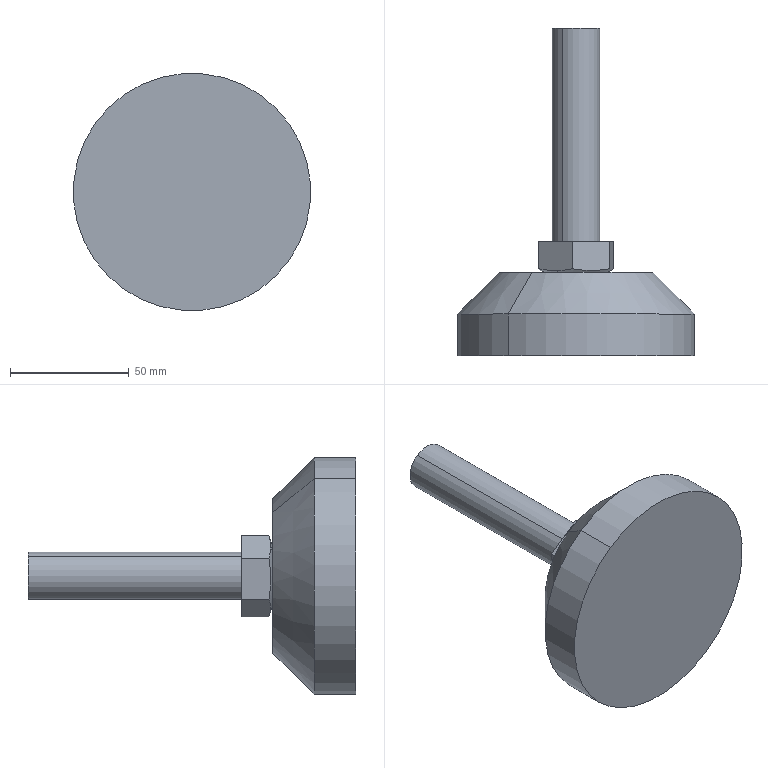Component | SolidWorks | 30-01A-1_Wheel-322-1_FBR100-20-322-1_pad1100-20-100pad1-322-1 | 1 solid | 23 faces | box 100 x 138 x 100 mm | volume 270529 mm3 | plane 11 | cylinder 8 | cone 4 | commonest cylinder face diameters 100 x2 57 x2 65 x2 20 x2
build123d program:
from build123d import *

# Parameters (mm, degrees)
SKETCH2_W          = 60
SKETCH2_H          = 60
CUT_EXTRUDE1_DEPTH = 14
SKETCH3_R          = 32.5
SKETCH3_R_2        = 28.5
CUT_EXTRUDE2_DEPTH = 0.1
SKETCH4_R          = 28.245
CUT_EXTRUDE3_DEPTH = 10


with BuildPart() as part:
    # Sketch1 → Revolve1 (revolve)
    with BuildSketch(Plane.XY, mode=Mode.PRIVATE) as revolve1_sk:
        Polygon((0, 148), (8.647, 148), (10, 146.647), (10, 48), (18.75, 48), (18.75, 37), (12, 35), (32.5, 35), (50, 17.5), (50, 0), (0, 0), align=None)
    revolve(revolve1_sk.sketch.rotate(Axis((0, 0, 0), (0, 1, 0)), 270), axis=Axis((0, 0, 0), (0, 1, 0)))

    # Sketch2 → Cut-Extrude1 (cut)
    with BuildSketch(Plane(origin=(0, 35, 0), x_dir=(-1, 0, 0), z_dir=(0, 1, 0))):
        Rectangle(SKETCH2_W, SKETCH2_H)
        Polygon((17.321, 0), (8.66, 15), (-8.66, 15), (-17.321, 0), (-8.66, -15), (8.66, -15), align=None, mode=Mode.SUBTRACT)
    extrude(amount=CUT_EXTRUDE1_DEPTH, mode=Mode.SUBTRACT)

    # Sketch3 → Cut-Extrude2 (cut)
    with BuildSketch(Plane(origin=(0, 35, 0), x_dir=(-1, 0, 0), z_dir=(0, 1, 0))):
        with Locations(Location((0, 0, 0), (0, 0, 90))):
            Circle(SKETCH3_R)
        with Locations(Location((0, 0, 0), (0, 0, 90))):
            Circle(SKETCH3_R_2, mode=Mode.SUBTRACT)
    extrude(amount=-CUT_EXTRUDE2_DEPTH, mode=Mode.SUBTRACT)

    # Sketch4 → Cut-Extrude3 (cut)
    with BuildSketch(Plane(origin=(0, 148, 0), x_dir=(1, 0, 0), z_dir=(0, 1, 0))):
        Circle(SKETCH4_R)
    extrude(amount=-CUT_EXTRUDE3_DEPTH, mode=Mode.SUBTRACT)


solid = part.part

# Placed as in the assembly
solid = solid.moved(Location((232.57, -660.845, -20), (180, 34.797, 180)))
STEP:
#1=CARTESIAN_POINT('',(9.886,-24.64,-1.838));
#2=VERTEX_POINT('',#1);
#3=CARTESIAN_POINT('',(8.426,-24.64,0.2633));
#4=VERTEX_POINT('',#3);
#5=CARTESIAN_POINT('',(9.156,-24.64,-0.7874));
#6=DIRECTION('',(0.,1.,-0.));
#7=DIRECTION('',(0.5707,0.,-0.8212));
#8=AXIS2_PLACEMENT_3D('',#5,#6,#7);
#9=CIRCLE('',#8,1.28);
#10=EDGE_CURVE('',#2,#4,#9,.T.);
#11=ORIENTED_EDGE('',*,*,#10,.F.);
#12=CARTESIAN_POINT('',(10.28,-25.329,-2.404));
#13=VERTEX_POINT('',#12);
#14=CARTESIAN_POINT('',(10.28,-25.329,-2.404));
#15=DIRECTION('',(0.4035,-0.7071,-0.5807));
#16=VECTOR('',#15,39.37);
#17=LINE('',#14,#16);
#18=EDGE_CURVE('',#2,#13,#17,.T.);
#19=ORIENTED_EDGE('',*,*,#18,.T.);
#20=CARTESIAN_POINT('',(8.033,-25.329,0.8291));
#21=VERTEX_POINT('',#20);
#22=CARTESIAN_POINT('',(9.156,-25.329,-0.7874));
#23=DIRECTION('',(0.,1.,-0.));
#24=DIRECTION('',(0.5707,0.,-0.8212));
#25=AXIS2_PLACEMENT_3D('',#22,#23,#24);
#26=CIRCLE('',#25,1.969);
#27=EDGE_CURVE('',#13,#21,#26,.T.);
#28=ORIENTED_EDGE('',*,*,#27,.T.);
#29=CARTESIAN_POINT('',(8.033,-25.329,0.8291));
#30=DIRECTION('',(-0.4035,-0.7071,0.5807));
#31=VECTOR('',#30,39.37);
#32=LINE('',#29,#31);
#33=EDGE_CURVE('',#4,#21,#32,.T.);
#34=ORIENTED_EDGE('',*,*,#33,.F.);
#35=EDGE_LOOP('',(#11,#19,#28,#34));
#36=FACE_OUTER_BOUND('',#35,.T.);
#37=CARTESIAN_POINT('',(9.156,-25.329,-0.7874));
#38=DIRECTION('',(-0.,-1.,0.));
#39=DIRECTION('',(-0.5707,0.,0.8212));
#40=AXIS2_PLACEMENT_3D('',#37,#38,#39);
#41=CONICAL_SURFACE('',#40,1.969,0.7854);
#42=ADVANCED_FACE('',(#36),#41,.T.);
#43=CARTESIAN_POINT('',(10.28,-26.018,-2.404));
#44=VERTEX_POINT('',#43);
#45=CARTESIAN_POINT('',(8.033,-26.018,0.8291));
#46=VERTEX_POINT('',#45);
#47=CARTESIAN_POINT('',(9.156,-26.018,-0.7874));
#48=DIRECTION('',(0.,1.,-0.));
#49=DIRECTION('',(0.5707,0.,-0.8212));
#50=AXIS2_PLACEMENT_3D('',#47,#48,#49);
#51=CIRCLE('',#50,1.969);
#52=EDGE_CURVE('',#44,#46,#51,.T.);
#53=ORIENTED_EDGE('',*,*,#52,.T.);
#54=CARTESIAN_POINT('',(8.033,-26.018,0.8291));
#55=DIRECTION('',(0.,1.,-0.));
#56=VECTOR('',#55,39.37);
#57=LINE('',#54,#56);
#58=EDGE_CURVE('',#46,#21,#57,.T.);
#59=ORIENTED_EDGE('',*,*,#58,.T.);
#60=ORIENTED_EDGE('',*,*,#27,.F.);
#61=CARTESIAN_POINT('',(10.28,-26.018,-2.404));
#62=DIRECTION('',(0.,1.,-0.));
#63=VECTOR('',#62,39.37);
#64=LINE('',#61,#63);
#65=EDGE_CURVE('',#44,#13,#64,.T.);
#66=ORIENTED_EDGE('',*,*,#65,.F.);
#67=EDGE_LOOP('',(#53,#59,#60,#66));
#68=FACE_OUTER_BOUND('',#67,.T.);
#69=CARTESIAN_POINT('',(9.156,-26.018,-0.7874));
#70=DIRECTION('',(0.,1.,-0.));
#71=DIRECTION('',(0.5707,0.,-0.8212));
#72=AXIS2_PLACEMENT_3D('',#69,#70,#71);
#73=CYLINDRICAL_SURFACE('',#72,1.969);
#74=ADVANCED_FACE('',(#68),#73,.T.);
#75=CARTESIAN_POINT('',(9.797,-24.643,-1.709));
#76=VERTEX_POINT('',#75);
#77=CARTESIAN_POINT('',(8.516,-24.643,0.134));
#78=VERTEX_POINT('',#77);
#79=CARTESIAN_POINT('',(9.156,-24.643,-0.7874));
#80=DIRECTION('',(0.,1.,-0.));
#81=DIRECTION('',(0.5707,0.,-0.8212));
#82=AXIS2_PLACEMENT_3D('',#79,#80,#81);
#83=CIRCLE('',#82,1.122);
#84=EDGE_CURVE('',#76,#78,#83,.T.);
#85=ORIENTED_EDGE('',*,*,#84,.T.);
#86=CARTESIAN_POINT('',(8.516,-24.64,0.134));
#87=VERTEX_POINT('',#86);
#88=CARTESIAN_POINT('',(8.516,-24.643,0.134));
#89=DIRECTION('',(0.,1.,-0.));
#90=VECTOR('',#89,39.37);
#91=LINE('',#88,#90);
#92=EDGE_CURVE('',#78,#87,#91,.T.);
#93=ORIENTED_EDGE('',*,*,#92,.T.);
#94=CARTESIAN_POINT('',(9.797,-24.64,-1.709));
#95=VERTEX_POINT('',#94);
#96=CARTESIAN_POINT('',(9.156,-24.64,-0.7874));
#97=DIRECTION('',(0.,1.,-0.));
#98=DIRECTION('',(0.5707,0.,-0.8212));
#99=AXIS2_PLACEMENT_3D('',#96,#97,#98);
#100=CIRCLE('',#99,1.122);
#101=EDGE_CURVE('',#95,#87,#100,.T.);
#102=ORIENTED_EDGE('',*,*,#101,.F.);
#103=CARTESIAN_POINT('',(9.797,-24.643,-1.709));
#104=DIRECTION('',(0.,1.,-0.));
#105=VECTOR('',#104,39.37);
#106=LINE('',#103,#105);
#107=EDGE_CURVE('',#76,#95,#106,.T.);
#108=ORIENTED_EDGE('',*,*,#107,.F.);
#109=EDGE_LOOP('',(#85,#93,#102,#108));
#110=FACE_OUTER_BOUND('',#109,.T.);
#111=CARTESIAN_POINT('',(9.156,-24.643,-0.7874));
#112=DIRECTION('',(0.,1.,-0.));
#113=DIRECTION('',(0.5707,0.,-0.8212));
#114=AXIS2_PLACEMENT_3D('',#111,#112,#113);
#115=CYLINDRICAL_SURFACE('',#114,1.122);
#116=ADVANCED_FACE('',(#110),#115,.T.);
#117=CARTESIAN_POINT('',(8.426,-24.643,0.2633));
#118=VERTEX_POINT('',#117);
#119=CARTESIAN_POINT('',(9.886,-24.643,-1.838));
#120=VERTEX_POINT('',#119);
#121=CARTESIAN_POINT('',(9.156,-24.643,-0.7874));
#122=DIRECTION('',(0.,1.,-0.));
#123=DIRECTION('',(0.5707,0.,-0.8212));
#124=AXIS2_PLACEMENT_3D('',#121,#122,#123);
#125=CIRCLE('',#124,1.28);
#126=EDGE_CURVE('',#118,#120,#125,.T.);
#127=ORIENTED_EDGE('',*,*,#126,.F.);
#128=CARTESIAN_POINT('',(8.426,-24.643,0.2633));
#129=DIRECTION('',(0.,1.,-0.));
#130=VECTOR('',#129,39.37);
#131=LINE('',#128,#130);
#132=EDGE_CURVE('',#118,#4,#131,.T.);
#133=ORIENTED_EDGE('',*,*,#132,.T.);
#134=CARTESIAN_POINT('',(9.156,-24.64,-0.7874));
#135=DIRECTION('',(0.,1.,-0.));
#136=DIRECTION('',(0.5707,0.,-0.8212));
#137=AXIS2_PLACEMENT_3D('',#134,#135,#136);
#138=CIRCLE('',#137,1.28);
#139=EDGE_CURVE('',#4,#2,#138,.T.);
#140=ORIENTED_EDGE('',*,*,#139,.T.);
#141=CARTESIAN_POINT('',(9.886,-24.643,-1.838));
#142=DIRECTION('',(0.,1.,-0.));
#143=VECTOR('',#142,39.37);
#144=LINE('',#141,#143);
#145=EDGE_CURVE('',#120,#2,#144,.T.);
#146=ORIENTED_EDGE('',*,*,#145,.F.);
#147=EDGE_LOOP('',(#127,#133,#140,#146));
#148=FACE_OUTER_BOUND('',#147,.T.);
#149=CARTESIAN_POINT('',(9.156,-24.643,-0.7874));
#150=DIRECTION('',(0.,1.,-0.));
#151=DIRECTION('',(0.5707,0.,-0.8212));
#152=AXIS2_PLACEMENT_3D('',#149,#150,#151);
#153=CYLINDRICAL_SURFACE('',#152,1.28);
#154=ADVANCED_FACE('',(#148),#153,.F.);
#155=CARTESIAN_POINT('',(9.426,-24.64,-1.175));
#156=VERTEX_POINT('',#155);
#157=CARTESIAN_POINT('',(8.887,-24.64,-0.3994));
#158=VERTEX_POINT('',#157);
#159=CARTESIAN_POINT('',(9.156,-24.64,-0.7874));
#160=DIRECTION('',(0.,1.,-0.));
#161=DIRECTION('',(0.5707,0.,-0.8212));
#162=AXIS2_PLACEMENT_3D('',#159,#160,#161);
#163=CIRCLE('',#162,0.4724);
#164=EDGE_CURVE('',#156,#158,#163,.T.);
#165=ORIENTED_EDGE('',*,*,#164,.T.);
#166=CARTESIAN_POINT('',(8.819,-24.605,-0.3024));
#167=VERTEX_POINT('',#166);
#168=CARTESIAN_POINT('',(8.887,-24.64,-0.3994));
#169=DIRECTION('',(-0.5471,0.2841,0.7874));
#170=VECTOR('',#169,39.37);
#171=LINE('',#168,#170);
#172=EDGE_CURVE('',#158,#167,#171,.T.);
#173=ORIENTED_EDGE('',*,*,#172,.T.);
#174=CARTESIAN_POINT('',(8.539,-24.577,-0.497));
#175=VERTEX_POINT('',#174);
#176=CARTESIAN_POINT('',(8.819,-24.605,-0.3024));
#177=CARTESIAN_POINT('',(8.773,-24.605,-0.335));
#178=CARTESIAN_POINT('',(8.726,-24.602,-0.3674));
#179=CARTESIAN_POINT('',(8.632,-24.593,-0.4323));
#180=CARTESIAN_POINT('',(8.586,-24.586,-0.4647));
#181=CARTESIAN_POINT('',(8.539,-24.577,-0.497));
#182=B_SPLINE_CURVE_WITH_KNOTS('',3,(#176,#177,#178,#179,#180,#181),.UNSPECIFIED.,.F.,.F.,(4,2,4),(0.02323,0.0276,0.03198),.UNSPECIFIED.);
#183=EDGE_CURVE('',#167,#175,#182,.T.);
#184=ORIENTED_EDGE('',*,*,#183,.T.);
#185=CARTESIAN_POINT('',(8.596,-24.577,-1.177));
#186=VERTEX_POINT('',#185);
#187=CARTESIAN_POINT('',(8.539,-24.577,-0.497));
#188=CARTESIAN_POINT('',(8.544,-24.586,-0.5536));
#189=CARTESIAN_POINT('',(8.549,-24.593,-0.6103));
#190=CARTESIAN_POINT('',(8.558,-24.602,-0.7235));
#191=CARTESIAN_POINT('',(8.568,-24.607,-0.8368));
#192=CARTESIAN_POINT('',(8.577,-24.602,-0.95));
#193=CARTESIAN_POINT('',(8.587,-24.593,-1.063));
#194=CARTESIAN_POINT('',(8.592,-24.586,-1.12));
#195=CARTESIAN_POINT('',(8.596,-24.577,-1.177));
#196=B_SPLINE_CURVE_WITH_KNOTS('',3,(#187,#188,#189,#190,#191,#192,#193,#194,#195),.UNSPECIFIED.,.F.,.F.,(4,2,1,2,4),(0.00000023,0.00433,0.00866,0.01299,0.01732),.UNSPECIFIED.);
#197=EDGE_CURVE('',#175,#186,#196,.T.);
#198=ORIENTED_EDGE('',*,*,#197,.T.);
#199=CARTESIAN_POINT('',(9.213,-24.577,-1.467));
#200=VERTEX_POINT('',#199);
#201=CARTESIAN_POINT('',(8.596,-24.577,-1.177));
#202=CARTESIAN_POINT('',(8.648,-24.586,-1.201));
#203=CARTESIAN_POINT('',(8.699,-24.593,-1.225));
#204=CARTESIAN_POINT('',(8.802,-24.602,-1.273));
#205=CARTESIAN_POINT('',(8.905,-24.607,-1.322));
#206=CARTESIAN_POINT('',(9.008,-24.602,-1.37));
#207=CARTESIAN_POINT('',(9.11,-24.593,-1.419));
#208=CARTESIAN_POINT('',(9.162,-24.586,-1.443));
#209=CARTESIAN_POINT('',(9.213,-24.577,-1.467));
#210=B_SPLINE_CURVE_WITH_KNOTS('',3,(#201,#202,#203,#204,#205,#206,#207,#208,#209),.UNSPECIFIED.,.F.,.F.,(4,2,1,2,4),(0.00000023,0.00433,0.00866,0.01299,0.01732),.UNSPECIFIED.);
#211=EDGE_CURVE('',#186,#200,#210,.T.);
#212=ORIENTED_EDGE('',*,*,#211,.T.);
#213=CARTESIAN_POINT('',(9.493,-24.605,-1.272));
#214=VERTEX_POINT('',#213);
#215=CARTESIAN_POINT('',(9.213,-24.577,-1.467));
#216=CARTESIAN_POINT('',(9.26,-24.586,-1.435));
#217=CARTESIAN_POINT('',(9.306,-24.593,-1.402));
#218=CARTESIAN_POINT('',(9.4,-24.602,-1.337));
#219=CARTESIAN_POINT('',(9.447,-24.605,-1.305));
#220=CARTESIAN_POINT('',(9.493,-24.605,-1.272));
#221=B_SPLINE_CURVE_WITH_KNOTS('',3,(#215,#216,#217,#218,#219,#220),.UNSPECIFIED.,.F.,.F.,(4,2,4),(0.03359,0.03796,0.04232),.UNSPECIFIED.);
#222=EDGE_CURVE('',#200,#214,#221,.T.);
#223=ORIENTED_EDGE('',*,*,#222,.T.);
#224=CARTESIAN_POINT('',(9.426,-24.64,-1.175));
#225=DIRECTION('',(0.5471,0.2841,-0.7874));
#226=VECTOR('',#225,39.37);
#227=LINE('',#224,#226);
#228=EDGE_CURVE('',#156,#214,#227,.T.);
#229=ORIENTED_EDGE('',*,*,#228,.F.);
#230=EDGE_LOOP('',(#165,#173,#184,#198,#212,#223,#229));
#231=FACE_OUTER_BOUND('',#230,.T.);
#232=CARTESIAN_POINT('',(9.156,-24.64,-0.7874));
#233=DIRECTION('',(0.,1.,-0.));
#234=DIRECTION('',(0.5707,0.,-0.8212));
#235=AXIS2_PLACEMENT_3D('',#232,#233,#234);
#236=CONICAL_SURFACE('',#235,0.4724,1.283);
#237=ADVANCED_FACE('',(#231),#236,.T.);
#238=CARTESIAN_POINT('',(9.381,-24.128,-1.111));
#239=VERTEX_POINT('',#238);
#240=CARTESIAN_POINT('',(8.932,-24.128,-0.4641));
#241=VERTEX_POINT('',#240);
#242=CARTESIAN_POINT('',(9.156,-24.128,-0.7874));
#243=DIRECTION('',(0.,1.,-0.));
#244=DIRECTION('',(0.5707,0.,-0.8212));
#245=AXIS2_PLACEMENT_3D('',#242,#243,#244);
#246=CIRCLE('',#245,0.3937);
#247=EDGE_CURVE('',#239,#241,#246,.T.);
#248=ORIENTED_EDGE('',*,*,#247,.T.);
#249=CARTESIAN_POINT('',(8.932,-20.584,-0.4641));
#250=VERTEX_POINT('',#249);
#251=CARTESIAN_POINT('',(8.932,-26.018,-0.4641));
#252=DIRECTION('',(0.,1.,-0.));
#253=VECTOR('',#252,39.37);
#254=LINE('',#251,#253);
#255=EDGE_CURVE('',#241,#250,#254,.T.);
#256=ORIENTED_EDGE('',*,*,#255,.T.);
#257=CARTESIAN_POINT('',(9.381,-20.584,-1.111));
#258=VERTEX_POINT('',#257);
#259=CARTESIAN_POINT('',(9.156,-20.584,-0.7874));
#260=DIRECTION('',(0.,1.,-0.));
#261=DIRECTION('',(0.5707,0.,-0.8212));
#262=AXIS2_PLACEMENT_3D('',#259,#260,#261);
#263=CIRCLE('',#262,0.3937);
#264=EDGE_CURVE('',#258,#250,#263,.T.);
#265=ORIENTED_EDGE('',*,*,#264,.F.);
#266=CARTESIAN_POINT('',(9.381,-26.018,-1.111));
#267=DIRECTION('',(0.,1.,-0.));
#268=VECTOR('',#267,39.37);
#269=LINE('',#266,#268);
#270=EDGE_CURVE('',#239,#258,#269,.T.);
#271=ORIENTED_EDGE('',*,*,#270,.F.);
#272=EDGE_LOOP('',(#248,#256,#265,#271));
#273=FACE_OUTER_BOUND('',#272,.T.);
#274=CARTESIAN_POINT('',(9.156,-26.018,-0.7874));
#275=DIRECTION('',(0.,1.,-0.));
#276=DIRECTION('',(0.5707,0.,-0.8212));
#277=AXIS2_PLACEMENT_3D('',#274,#275,#276);
#278=CYLINDRICAL_SURFACE('',#277,0.3937);
#279=ADVANCED_FACE('',(#273),#278,.T.);
#280=ORIENTED_EDGE('',*,*,#255,.F.);
#281=CARTESIAN_POINT('',(9.156,-24.128,-0.7874));
#282=DIRECTION('',(0.,1.,-0.));
#283=DIRECTION('',(0.5707,0.,-0.8212));
#284=AXIS2_PLACEMENT_3D('',#281,#282,#283);
#285=CIRCLE('',#284,0.3937);
#286=EDGE_CURVE('',#241,#239,#285,.T.);
#287=ORIENTED_EDGE('',*,*,#286,.T.);
#288=ORIENTED_EDGE('',*,*,#270,.T.);
#289=CARTESIAN_POINT('',(9.156,-20.584,-0.7874));
#290=DIRECTION('',(0.,1.,-0.));
#291=DIRECTION('',(0.5707,0.,-0.8212));
#292=AXIS2_PLACEMENT_3D('',#289,#290,#291);
#293=CIRCLE('',#292,0.3937);
#294=EDGE_CURVE('',#250,#258,#293,.T.);
#295=ORIENTED_EDGE('',*,*,#294,.F.);
#296=EDGE_LOOP('',(#280,#287,#288,#295));
#297=FACE_OUTER_BOUND('',#296,.T.);
#298=CARTESIAN_POINT('',(9.156,-26.018,-0.7874));
#299=DIRECTION('',(0.,1.,-0.));
#300=DIRECTION('',(0.5707,0.,-0.8212));
#301=AXIS2_PLACEMENT_3D('',#298,#299,#300);
#302=CYLINDRICAL_SURFACE('',#301,0.3937);
#303=ADVANCED_FACE('',(#297),#302,.T.);
#304=ORIENTED_EDGE('',*,*,#164,.F.);
#305=CARTESIAN_POINT('',(9.156,-24.64,-0.7874));
#306=DIRECTION('',(0.,1.,-0.));
#307=DIRECTION('',(0.5707,0.,-0.8212));
#308=AXIS2_PLACEMENT_3D('',#305,#306,#307);
#309=CIRCLE('',#308,0.4724);
#310=EDGE_CURVE('',#158,#156,#309,.T.);
#311=ORIENTED_EDGE('',*,*,#310,.F.);
#312=EDGE_LOOP('',(#304,#311));
#313=FACE_BOUND('',#312,.T.);
#314=ORIENTED_EDGE('',*,*,#101,.T.);
#315=CARTESIAN_POINT('',(9.156,-24.64,-0.7874));
#316=DIRECTION('',(0.,1.,-0.));
#317=DIRECTION('',(0.5707,0.,-0.8212));
#318=AXIS2_PLACEMENT_3D('',#315,#316,#317);
#319=CIRCLE('',#318,1.122);
#320=EDGE_CURVE('',#87,#95,#319,.T.);
#321=ORIENTED_EDGE('',*,*,#320,.T.);
#322=EDGE_LOOP('',(#314,#321));
#323=FACE_OUTER_BOUND('',#322,.T.);
#324=CARTESIAN_POINT('',(8.768,-24.64,-1.057));
#325=DIRECTION('',(-0.,-1.,0.));
#326=DIRECTION('',(-0.5707,0.,0.8212));
#327=AXIS2_PLACEMENT_3D('',#324,#325,#326);
#328=PLANE('',#327);
#329=ADVANCED_FACE('',(#313,#323),#328,.F.);
#330=ORIENTED_EDGE('',*,*,#172,.F.);
#331=ORIENTED_EDGE('',*,*,#310,.T.);
#332=ORIENTED_EDGE('',*,*,#228,.T.);
#333=CARTESIAN_POINT('',(9.773,-24.577,-1.078));
#334=VERTEX_POINT('',#333);
#335=CARTESIAN_POINT('',(9.493,-24.605,-1.272));
#336=CARTESIAN_POINT('',(9.54,-24.605,-1.24));
#337=CARTESIAN_POINT('',(9.587,-24.602,-1.208));
#338=CARTESIAN_POINT('',(9.68,-24.593,-1.143));
#339=CARTESIAN_POINT('',(9.727,-24.586,-1.11));
#340=CARTESIAN_POINT('',(9.773,-24.577,-1.078));
#341=B_SPLINE_CURVE_WITH_KNOTS('',3,(#335,#336,#337,#338,#339,#340),.UNSPECIFIED.,.F.,.F.,(4,2,4),(0.04232,0.04667,0.05102),.UNSPECIFIED.);
#342=EDGE_CURVE('',#214,#334,#341,.T.);
#343=ORIENTED_EDGE('',*,*,#342,.T.);
#344=CARTESIAN_POINT('',(9.716,-24.577,-0.3983));
#345=VERTEX_POINT('',#344);
#346=CARTESIAN_POINT('',(9.773,-24.577,-1.078));
#347=CARTESIAN_POINT('',(9.769,-24.586,-1.021));
#348=CARTESIAN_POINT('',(9.764,-24.593,-0.9645));
#349=CARTESIAN_POINT('',(9.754,-24.602,-0.8513));
#350=CARTESIAN_POINT('',(9.745,-24.607,-0.738));
#351=CARTESIAN_POINT('',(9.735,-24.602,-0.6248));
#352=CARTESIAN_POINT('',(9.726,-24.593,-0.5115));
#353=CARTESIAN_POINT('',(9.721,-24.586,-0.4549));
#354=CARTESIAN_POINT('',(9.716,-24.577,-0.3983));
#355=B_SPLINE_CURVE_WITH_KNOTS('',3,(#346,#347,#348,#349,#350,#351,#352,#353,#354),.UNSPECIFIED.,.F.,.F.,(4,2,1,2,4),(0.00000023,0.00433,0.00866,0.01299,0.01732),.UNSPECIFIED.);
#356=EDGE_CURVE('',#334,#345,#355,.T.);
#357=ORIENTED_EDGE('',*,*,#356,.T.);
#358=CARTESIAN_POINT('',(9.099,-24.577,-0.1079));
#359=VERTEX_POINT('',#358);
#360=CARTESIAN_POINT('',(9.716,-24.577,-0.3983));
#361=CARTESIAN_POINT('',(9.665,-24.586,-0.3741));
#362=CARTESIAN_POINT('',(9.613,-24.593,-0.3499));
#363=CARTESIAN_POINT('',(9.511,-24.602,-0.3015));
#364=CARTESIAN_POINT('',(9.408,-24.607,-0.2531));
#365=CARTESIAN_POINT('',(9.305,-24.602,-0.2047));
#366=CARTESIAN_POINT('',(9.202,-24.593,-0.1563));
#367=CARTESIAN_POINT('',(9.151,-24.586,-0.1321));
#368=CARTESIAN_POINT('',(9.099,-24.577,-0.1079));
#369=B_SPLINE_CURVE_WITH_KNOTS('',3,(#360,#361,#362,#363,#364,#365,#366,#367,#368),.UNSPECIFIED.,.F.,.F.,(4,2,1,2,4),(0.00000023,0.00433,0.00866,0.01299,0.01732),.UNSPECIFIED.);
#370=EDGE_CURVE('',#345,#359,#369,.T.);
#371=ORIENTED_EDGE('',*,*,#370,.T.);
#372=CARTESIAN_POINT('',(9.099,-24.577,-0.1079));
#373=CARTESIAN_POINT('',(9.053,-24.586,-0.1402));
#374=CARTESIAN_POINT('',(9.006,-24.593,-0.1727));
#375=CARTESIAN_POINT('',(8.913,-24.602,-0.2377));
#376=CARTESIAN_POINT('',(8.866,-24.605,-0.2701));
#377=CARTESIAN_POINT('',(8.819,-24.605,-0.3024));
#378=B_SPLINE_CURVE_WITH_KNOTS('',3,(#372,#373,#374,#375,#376,#377),.UNSPECIFIED.,.F.,.F.,(4,2,4),(0.01452,0.01887,0.02323),.UNSPECIFIED.);
#379=EDGE_CURVE('',#359,#167,#378,.T.);
#380=ORIENTED_EDGE('',*,*,#379,.T.);
#381=EDGE_LOOP('',(#330,#331,#332,#343,#357,#371,#380));
#382=FACE_OUTER_BOUND('',#381,.T.);
#383=CARTESIAN_POINT('',(9.156,-24.64,-0.7874));
#384=DIRECTION('',(0.,1.,-0.));
#385=DIRECTION('',(0.5707,0.,-0.8212));
#386=AXIS2_PLACEMENT_3D('',#383,#384,#385);
#387=CONICAL_SURFACE('',#386,0.4724,1.283);
#388=ADVANCED_FACE('',(#382),#387,.T.);
#389=CARTESIAN_POINT('',(9.099,-24.128,-0.1079));
#390=VERTEX_POINT('',#389);
#391=CARTESIAN_POINT('',(9.099,-24.088,-0.1079));
#392=DIRECTION('',(-0.,-1.,0.));
#393=VECTOR('',#392,39.37);
#394=LINE('',#391,#393);
#395=EDGE_CURVE('',#390,#359,#394,.T.);
#396=ORIENTED_EDGE('',*,*,#395,.T.);
#397=ORIENTED_EDGE('',*,*,#370,.F.);
#398=CARTESIAN_POINT('',(9.716,-24.128,-0.3983));
#399=VERTEX_POINT('',#398);
#400=CARTESIAN_POINT('',(9.716,-24.088,-0.3983));
#401=DIRECTION('',(-0.,-1.,0.));
#402=VECTOR('',#401,39.37);
#403=LINE('',#400,#402);
#404=EDGE_CURVE('',#399,#345,#403,.T.);
#405=ORIENTED_EDGE('',*,*,#404,.F.);
#406=CARTESIAN_POINT('',(9.23,-24.128,-0.1692));
#407=DIRECTION('',(0.9048,-0.,-0.4258));
#408=VECTOR('',#407,39.37);
#409=LINE('',#406,#408);
#410=EDGE_CURVE('',#390,#399,#409,.T.);
#411=ORIENTED_EDGE('',*,*,#410,.F.);
#412=EDGE_LOOP('',(#396,#397,#405,#411));
#413=FACE_OUTER_BOUND('',#412,.T.);
#414=CARTESIAN_POINT('',(9.099,-24.088,-0.1079));
#415=DIRECTION('',(-0.4258,0.,-0.9048));
#416=DIRECTION('',(-0.9048,0.,0.4258));
#417=AXIS2_PLACEMENT_3D('',#414,#415,#416);
#418=PLANE('',#417);
#419=ADVANCED_FACE('',(#413),#418,.F.);
#420=ORIENTED_EDGE('',*,*,#404,.T.);
#421=ORIENTED_EDGE('',*,*,#356,.F.);
#422=CARTESIAN_POINT('',(9.773,-24.128,-1.078));
#423=VERTEX_POINT('',#422);
#424=CARTESIAN_POINT('',(9.773,-24.088,-1.078));
#425=DIRECTION('',(-0.,-1.,0.));
#426=VECTOR('',#425,39.37);
#427=LINE('',#424,#426);
#428=EDGE_CURVE('',#423,#334,#427,.T.);
#429=ORIENTED_EDGE('',*,*,#428,.F.);
#430=CARTESIAN_POINT('',(9.761,-24.128,-0.9342));
#431=DIRECTION('',(0.0836,-0.,-0.9965));
#432=VECTOR('',#431,39.37);
#433=LINE('',#430,#432);
#434=EDGE_CURVE('',#399,#423,#433,.T.);
#435=ORIENTED_EDGE('',*,*,#434,.F.);
#436=EDGE_LOOP('',(#420,#421,#429,#435));
#437=FACE_OUTER_BOUND('',#436,.T.);
#438=CARTESIAN_POINT('',(9.716,-24.088,-0.3983));
#439=DIRECTION('',(-0.9965,0.,-0.0836));
#440=DIRECTION('',(-0.0836,0.,0.9965));
#441=AXIS2_PLACEMENT_3D('',#438,#439,#440);
#442=PLANE('',#441);
#443=ADVANCED_FACE('',(#437),#442,.F.);
#444=ORIENTED_EDGE('',*,*,#428,.T.);
#445=ORIENTED_EDGE('',*,*,#342,.F.);
#446=ORIENTED_EDGE('',*,*,#222,.F.);
#447=CARTESIAN_POINT('',(9.213,-24.128,-1.467));
#448=VERTEX_POINT('',#447);
#449=CARTESIAN_POINT('',(9.213,-24.088,-1.467));
#450=DIRECTION('',(-0.,-1.,0.));
#451=VECTOR('',#450,39.37);
#452=LINE('',#449,#451);
#453=EDGE_CURVE('',#448,#200,#452,.T.);
#454=ORIENTED_EDGE('',*,*,#453,.F.);
#455=CARTESIAN_POINT('',(9.17,-24.128,-1.497));
#456=DIRECTION('',(-0.8212,0.,-0.5707));
#457=VECTOR('',#456,39.37);
#458=LINE('',#455,#457);
#459=EDGE_CURVE('',#423,#448,#458,.T.);
#460=ORIENTED_EDGE('',*,*,#459,.F.);
#461=EDGE_LOOP('',(#444,#445,#446,#454,#460));
#462=FACE_OUTER_BOUND('',#461,.T.);
#463=CARTESIAN_POINT('',(9.773,-24.088,-1.078));
#464=DIRECTION('',(-0.5707,0.,0.8212));
#465=DIRECTION('',(0.8212,-0.,0.5707));
#466=AXIS2_PLACEMENT_3D('',#463,#464,#465);
#467=PLANE('',#466);
#468=ADVANCED_FACE('',(#462),#467,.F.);
#469=ORIENTED_EDGE('',*,*,#453,.T.);
#470=ORIENTED_EDGE('',*,*,#211,.F.);
#471=CARTESIAN_POINT('',(8.596,-24.128,-1.177));
#472=VERTEX_POINT('',#471);
#473=CARTESIAN_POINT('',(8.596,-24.088,-1.177));
#474=DIRECTION('',(-0.,-1.,0.));
#475=VECTOR('',#474,39.37);
#476=LINE('',#473,#475);
#477=EDGE_CURVE('',#472,#186,#476,.T.);
#478=ORIENTED_EDGE('',*,*,#477,.F.);
#479=CARTESIAN_POINT('',(8.727,-24.128,-1.238));
#480=DIRECTION('',(-0.9048,0.,0.4258));
#481=VECTOR('',#480,39.37);
#482=LINE('',#479,#481);
#483=EDGE_CURVE('',#448,#472,#482,.T.);
#484=ORIENTED_EDGE('',*,*,#483,.F.);
#485=EDGE_LOOP('',(#469,#470,#478,#484));
#486=FACE_OUTER_BOUND('',#485,.T.);
#487=CARTESIAN_POINT('',(9.213,-24.088,-1.467));
#488=DIRECTION('',(0.4258,-0.,0.9048));
#489=DIRECTION('',(0.9048,-0.,-0.4258));
#490=AXIS2_PLACEMENT_3D('',#487,#488,#489);
#491=PLANE('',#490);
#492=ADVANCED_FACE('',(#486),#491,.F.);
#493=ORIENTED_EDGE('',*,*,#477,.T.);
#494=ORIENTED_EDGE('',*,*,#197,.F.);
#495=CARTESIAN_POINT('',(8.539,-24.128,-0.497));
#496=VERTEX_POINT('',#495);
#497=CARTESIAN_POINT('',(8.539,-24.088,-0.497));
#498=DIRECTION('',(-0.,-1.,0.));
#499=VECTOR('',#498,39.37);
#500=LINE('',#497,#499);
#501=EDGE_CURVE('',#496,#175,#500,.T.);
#502=ORIENTED_EDGE('',*,*,#501,.F.);
#503=CARTESIAN_POINT('',(8.584,-24.128,-1.033));
#504=DIRECTION('',(-0.0836,0.,0.9965));
#505=VECTOR('',#504,39.37);
#506=LINE('',#503,#505);
#507=EDGE_CURVE('',#472,#496,#506,.T.);
#508=ORIENTED_EDGE('',*,*,#507,.F.);
#509=EDGE_LOOP('',(#493,#494,#502,#508));
#510=FACE_OUTER_BOUND('',#509,.T.);
#511=CARTESIAN_POINT('',(8.596,-24.088,-1.177));
#512=DIRECTION('',(0.9965,-0.,0.0836));
#513=DIRECTION('',(0.0836,-0.,-0.9965));
#514=AXIS2_PLACEMENT_3D('',#511,#512,#513);
#515=PLANE('',#514);
#516=ADVANCED_FACE('',(#510),#515,.F.);
#517=ORIENTED_EDGE('',*,*,#501,.T.);
#518=ORIENTED_EDGE('',*,*,#183,.F.);
#519=ORIENTED_EDGE('',*,*,#379,.F.);
#520=ORIENTED_EDGE('',*,*,#395,.F.);
#521=CARTESIAN_POINT('',(8.496,-24.128,-0.5271));
#522=DIRECTION('',(0.8212,-0.,0.5707));
#523=VECTOR('',#522,39.37);
#524=LINE('',#521,#523);
#525=EDGE_CURVE('',#496,#390,#524,.T.);
#526=ORIENTED_EDGE('',*,*,#525,.F.);
#527=EDGE_LOOP('',(#517,#518,#519,#520,#526));
#528=FACE_OUTER_BOUND('',#527,.T.);
#529=CARTESIAN_POINT('',(8.539,-24.088,-0.497));
#530=DIRECTION('',(0.5707,-0.,-0.8212));
#531=DIRECTION('',(-0.8212,0.,-0.5707));
#532=AXIS2_PLACEMENT_3D('',#529,#530,#531);
#533=PLANE('',#532);
#534=ADVANCED_FACE('',(#528),#533,.F.);
#535=ORIENTED_EDGE('',*,*,#525,.T.);
#536=ORIENTED_EDGE('',*,*,#410,.T.);
#537=ORIENTED_EDGE('',*,*,#434,.T.);
#538=ORIENTED_EDGE('',*,*,#459,.T.);
#539=ORIENTED_EDGE('',*,*,#483,.T.);
#540=ORIENTED_EDGE('',*,*,#507,.T.);
#541=EDGE_LOOP('',(#535,#536,#537,#538,#539,#540));
#542=FACE_OUTER_BOUND('',#541,.T.);
#543=ORIENTED_EDGE('',*,*,#247,.F.);
#544=ORIENTED_EDGE('',*,*,#286,.F.);
#545=EDGE_LOOP('',(#543,#544));
#546=FACE_BOUND('',#545,.T.);
#547=CARTESIAN_POINT('',(8.833,-24.128,-1.012));
#548=DIRECTION('',(-0.,-1.,0.));
#549=DIRECTION('',(-0.5707,0.,0.8212));
#550=AXIS2_PLACEMENT_3D('',#547,#548,#549);
#551=PLANE('',#550);
#552=ADVANCED_FACE('',(#542,#546),#551,.F.);
#553=ORIENTED_EDGE('',*,*,#132,.F.);
#554=CARTESIAN_POINT('',(9.156,-24.643,-0.7874));
#555=DIRECTION('',(0.,1.,-0.));
#556=DIRECTION('',(0.5707,0.,-0.8212));
#557=AXIS2_PLACEMENT_3D('',#554,#555,#556);
#558=CIRCLE('',#557,1.28);
#559=EDGE_CURVE('',#120,#118,#558,.T.);
#560=ORIENTED_EDGE('',*,*,#559,.F.);
#561=ORIENTED_EDGE('',*,*,#145,.T.);
#562=ORIENTED_EDGE('',*,*,#10,.T.);
#563=EDGE_LOOP('',(#553,#560,#561,#562));
#564=FACE_OUTER_BOUND('',#563,.T.);
#565=CARTESIAN_POINT('',(9.156,-24.643,-0.7874));
#566=DIRECTION('',(0.,1.,-0.));
#567=DIRECTION('',(0.5707,0.,-0.8212));
#568=AXIS2_PLACEMENT_3D('',#565,#566,#567);
#569=CYLINDRICAL_SURFACE('',#568,1.28);
#570=ADVANCED_FACE('',(#564),#569,.F.);
#571=ORIENTED_EDGE('',*,*,#84,.F.);
#572=CARTESIAN_POINT('',(9.156,-24.643,-0.7874));
#573=DIRECTION('',(0.,1.,-0.));
#574=DIRECTION('',(0.5707,0.,-0.8212));
#575=AXIS2_PLACEMENT_3D('',#572,#573,#574);
#576=CIRCLE('',#575,1.122);
#577=EDGE_CURVE('',#78,#76,#576,.T.);
#578=ORIENTED_EDGE('',*,*,#577,.F.);
#579=EDGE_LOOP('',(#571,#578));
#580=FACE_BOUND('',#579,.T.);
#581=ORIENTED_EDGE('',*,*,#559,.T.);
#582=ORIENTED_EDGE('',*,*,#126,.T.);
#583=EDGE_LOOP('',(#581,#582));
#584=FACE_OUTER_BOUND('',#583,.T.);
#585=CARTESIAN_POINT('',(9.156,-24.643,-0.7874));
#586=DIRECTION('',(0.,1.,-0.));
#587=DIRECTION('',(0.5707,-0.,-0.8212));
#588=AXIS2_PLACEMENT_3D('',#585,#586,#587);
#589=PLANE('',#588);
#590=ADVANCED_FACE('',(#580,#584),#589,.T.);
#591=ORIENTED_EDGE('',*,*,#92,.F.);
#592=ORIENTED_EDGE('',*,*,#577,.T.);
#593=ORIENTED_EDGE('',*,*,#107,.T.);
#594=ORIENTED_EDGE('',*,*,#320,.F.);
#595=EDGE_LOOP('',(#591,#592,#593,#594));
#596=FACE_OUTER_BOUND('',#595,.T.);
#597=CARTESIAN_POINT('',(9.156,-24.643,-0.7874));
#598=DIRECTION('',(0.,1.,-0.));
#599=DIRECTION('',(0.5707,0.,-0.8212));
#600=AXIS2_PLACEMENT_3D('',#597,#598,#599);
#601=CYLINDRICAL_SURFACE('',#600,1.122);
#602=ADVANCED_FACE('',(#596),#601,.T.);
#603=ORIENTED_EDGE('',*,*,#52,.F.);
#604=CARTESIAN_POINT('',(9.156,-26.018,-0.7874));
#605=DIRECTION('',(0.,1.,-0.));
#606=DIRECTION('',(0.5707,0.,-0.8212));
#607=AXIS2_PLACEMENT_3D('',#604,#605,#606);
#608=CIRCLE('',#607,1.969);
#609=EDGE_CURVE('',#46,#44,#608,.T.);
#610=ORIENTED_EDGE('',*,*,#609,.F.);
#611=EDGE_LOOP('',(#603,#610));
#612=FACE_OUTER_BOUND('',#611,.T.);
#613=CARTESIAN_POINT('',(7.54,-26.018,-1.911));
#614=DIRECTION('',(0.,1.,-0.));
#615=DIRECTION('',(0.5707,-0.,-0.8212));
#616=AXIS2_PLACEMENT_3D('',#613,#614,#615);
#617=PLANE('',#616);
#618=ADVANCED_FACE('',(#612),#617,.F.);
#619=ORIENTED_EDGE('',*,*,#58,.F.);
#620=ORIENTED_EDGE('',*,*,#609,.T.);
#621=ORIENTED_EDGE('',*,*,#65,.T.);
#622=CARTESIAN_POINT('',(9.156,-25.329,-0.7874));
#623=DIRECTION('',(0.,1.,-0.));
#624=DIRECTION('',(0.5707,0.,-0.8212));
#625=AXIS2_PLACEMENT_3D('',#622,#623,#624);
#626=CIRCLE('',#625,1.969);
#627=EDGE_CURVE('',#21,#13,#626,.T.);
#628=ORIENTED_EDGE('',*,*,#627,.F.);
#629=EDGE_LOOP('',(#619,#620,#621,#628));
#630=FACE_OUTER_BOUND('',#629,.T.);
#631=CARTESIAN_POINT('',(9.156,-26.018,-0.7874));
#632=DIRECTION('',(0.,1.,-0.));
#633=DIRECTION('',(0.5707,0.,-0.8212));
#634=AXIS2_PLACEMENT_3D('',#631,#632,#633);
#635=CYLINDRICAL_SURFACE('',#634,1.969);
#636=ADVANCED_FACE('',(#630),#635,.T.);
#637=ORIENTED_EDGE('',*,*,#18,.F.);
#638=ORIENTED_EDGE('',*,*,#139,.F.);
#639=ORIENTED_EDGE('',*,*,#33,.T.);
#640=ORIENTED_EDGE('',*,*,#627,.T.);
#641=EDGE_LOOP('',(#637,#638,#639,#640));
#642=FACE_OUTER_BOUND('',#641,.T.);
#643=CARTESIAN_POINT('',(9.156,-25.329,-0.7874));
#644=DIRECTION('',(-0.,-1.,0.));
#645=DIRECTION('',(-0.5707,0.,0.8212));
#646=AXIS2_PLACEMENT_3D('',#643,#644,#645);
#647=CONICAL_SURFACE('',#646,1.969,0.7854);
#648=ADVANCED_FACE('',(#642),#647,.T.);
#649=ORIENTED_EDGE('',*,*,#264,.T.);
#650=ORIENTED_EDGE('',*,*,#294,.T.);
#651=EDGE_LOOP('',(#649,#650));
#652=FACE_OUTER_BOUND('',#651,.T.);
#653=CARTESIAN_POINT('',(9.156,-20.584,-0.7874));
#654=DIRECTION('',(0.,1.,-0.));
#655=DIRECTION('',(0.5707,-0.,-0.8212));
#656=AXIS2_PLACEMENT_3D('',#653,#654,#655);
#657=PLANE('',#656);
#658=ADVANCED_FACE('',(#652),#657,.T.);
#659=CLOSED_SHELL('',(#42,#74,#116,#154,#237,#279,#303,#329,#388,#419,#443,#468,#492,#516,#534,#552,#570,#590,#602,#618,#636,#648,#658));
#660=MANIFOLD_SOLID_BREP('',#659);
#661=CARTESIAN_POINT('',(0.,0.,0.));
#662=DIRECTION('',(0.,0.,1.));
#663=DIRECTION('',(1.,0.,0.));
#664=AXIS2_PLACEMENT_3D('',#661,#662,#663);
#665=(LENGTH_UNIT()NAMED_UNIT(*)SI_UNIT($,.METRE.));
#666=LENGTH_MEASURE_WITH_UNIT(LENGTH_MEASURE(0.0254),#665);
#667=DIMENSIONAL_EXPONENTS(1.,0.,0.,0.,0.,0.,0.);
#668=(CONVERSION_BASED_UNIT('',#666)LENGTH_UNIT()NAMED_UNIT(#667));
#669=UNCERTAINTY_MEASURE_WITH_UNIT(LENGTH_MEASURE(0.00001),#668,'','');
#670=(NAMED_UNIT(*)PLANE_ANGLE_UNIT()SI_UNIT($,.RADIAN.));
#671=(NAMED_UNIT(*)SI_UNIT($,.STERADIAN.)SOLID_ANGLE_UNIT());
#672=(GEOMETRIC_REPRESENTATION_CONTEXT(3)GLOBAL_UNCERTAINTY_ASSIGNED_CONTEXT((#669))GLOBAL_UNIT_ASSIGNED_CONTEXT((#668,#670,#671))REPRESENTATION_CONTEXT('',''));
#673=ADVANCED_BREP_SHAPE_REPRESENTATION('',(#660,#664),#672);
#674=COLOUR_RGB('',0.7922,0.8196,0.9333);
#675=FILL_AREA_STYLE_COLOUR('',#674);
#676=FILL_AREA_STYLE('',(#675));
#677=SURFACE_STYLE_FILL_AREA(#676);
#678=SURFACE_SIDE_STYLE('',(#677));
#679=SURFACE_STYLE_USAGE(.BOTH.,#678);
#680=PRESENTATION_STYLE_ASSIGNMENT((#679));
#681=STYLED_ITEM('',(#680),#660);
#682=(LENGTH_UNIT()NAMED_UNIT(*)SI_UNIT($,.METRE.));
#683=LENGTH_MEASURE_WITH_UNIT(LENGTH_MEASURE(0.0254),#682);
#684=DIMENSIONAL_EXPONENTS(1.,0.,0.,0.,0.,0.,0.);
#685=(CONVERSION_BASED_UNIT('',#683)LENGTH_UNIT()NAMED_UNIT(#684));
#686=UNCERTAINTY_MEASURE_WITH_UNIT(LENGTH_MEASURE(0.00001),#685,'','');
#687=(NAMED_UNIT(*)PLANE_ANGLE_UNIT()SI_UNIT($,.RADIAN.));
#688=(NAMED_UNIT(*)SI_UNIT($,.STERADIAN.)SOLID_ANGLE_UNIT());
#689=(GEOMETRIC_REPRESENTATION_CONTEXT(3)GLOBAL_UNCERTAINTY_ASSIGNED_CONTEXT((#686))GLOBAL_UNIT_ASSIGNED_CONTEXT((#685,#687,#688))REPRESENTATION_CONTEXT('',''));
#690=MECHANICAL_DESIGN_GEOMETRIC_PRESENTATION_REPRESENTATION('',(#681),#689);
#691=PRESENTATION_LAYER_ASSIGNMENT('','',(#681));